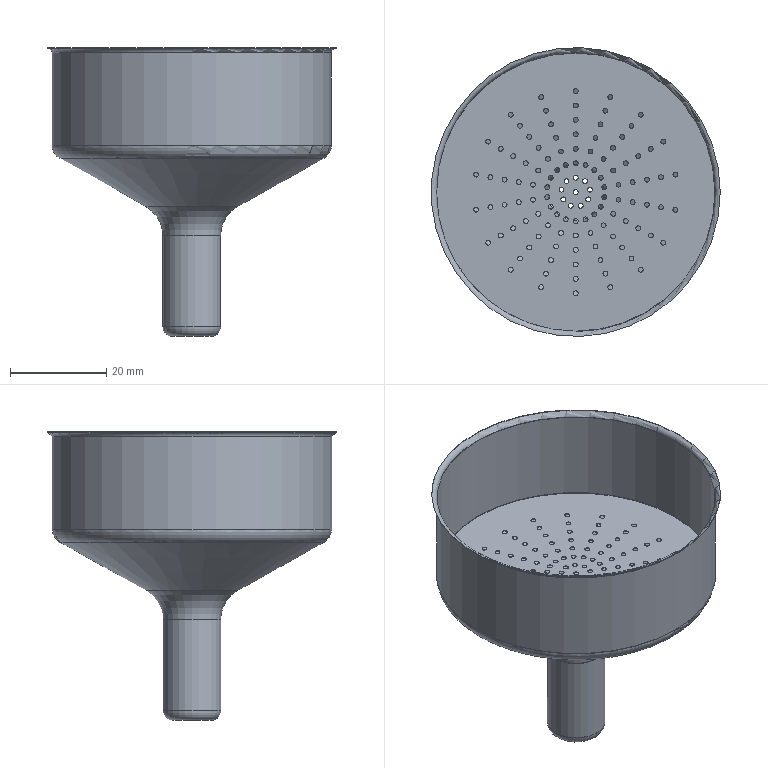Component | NX | MODEL24 | 1 solid | 136 faces | volume 1042 mm3 | cylinder 124 | torus 8 | plane 2 | cone 2 | commonest cylinder face diameters 1 x118 11.8 x1 8 x1 12 x1 58 x1 60 x1 57.8 x1